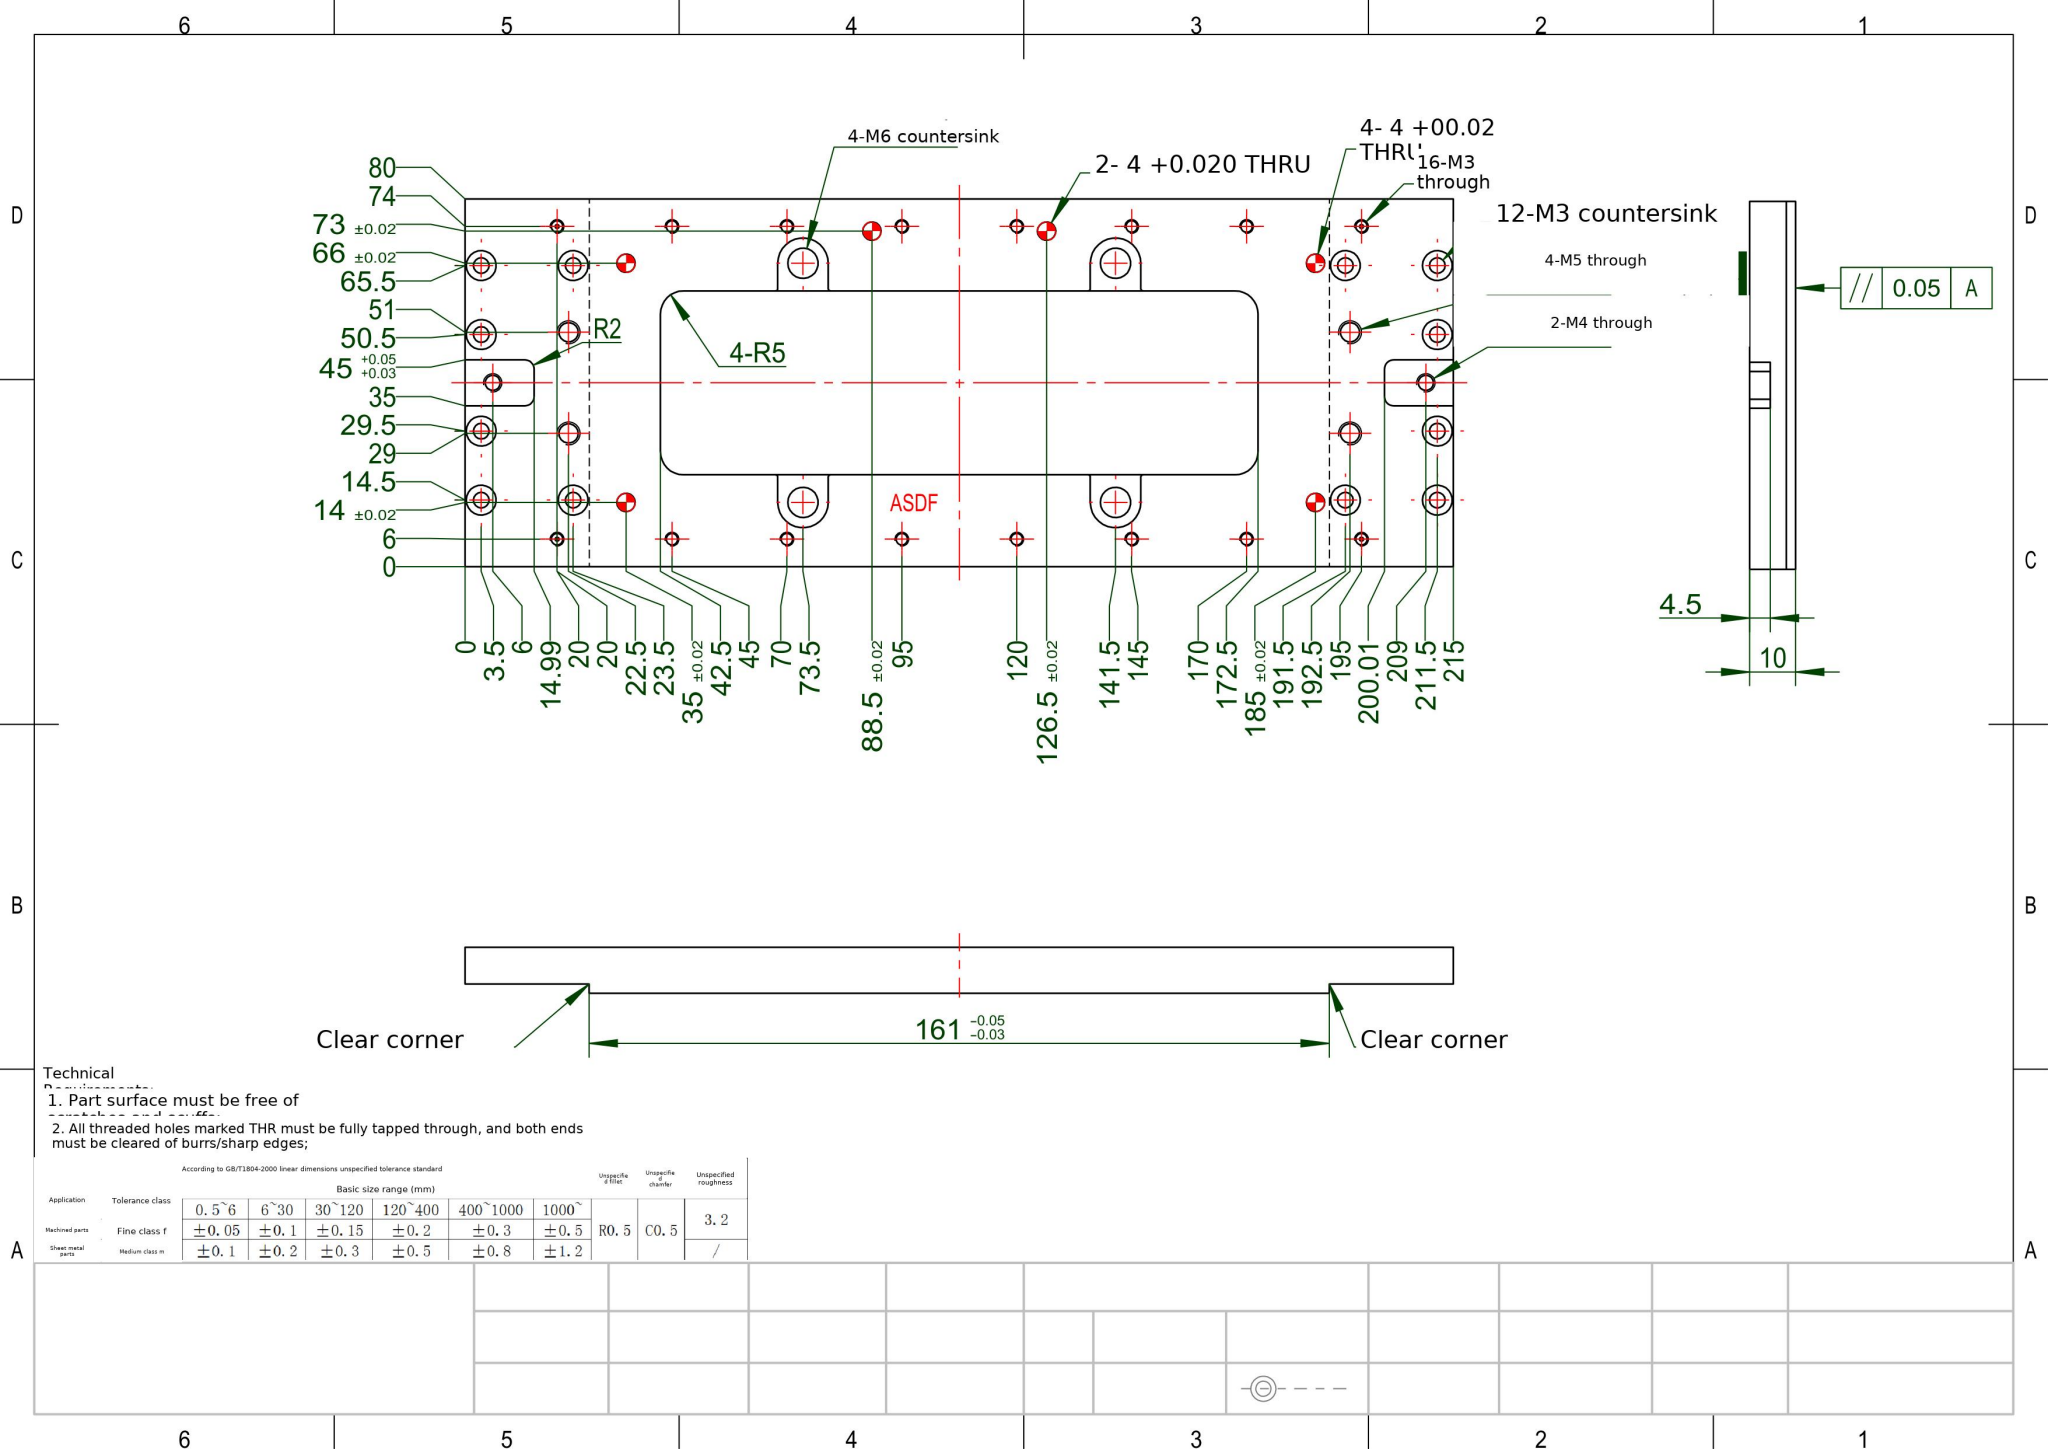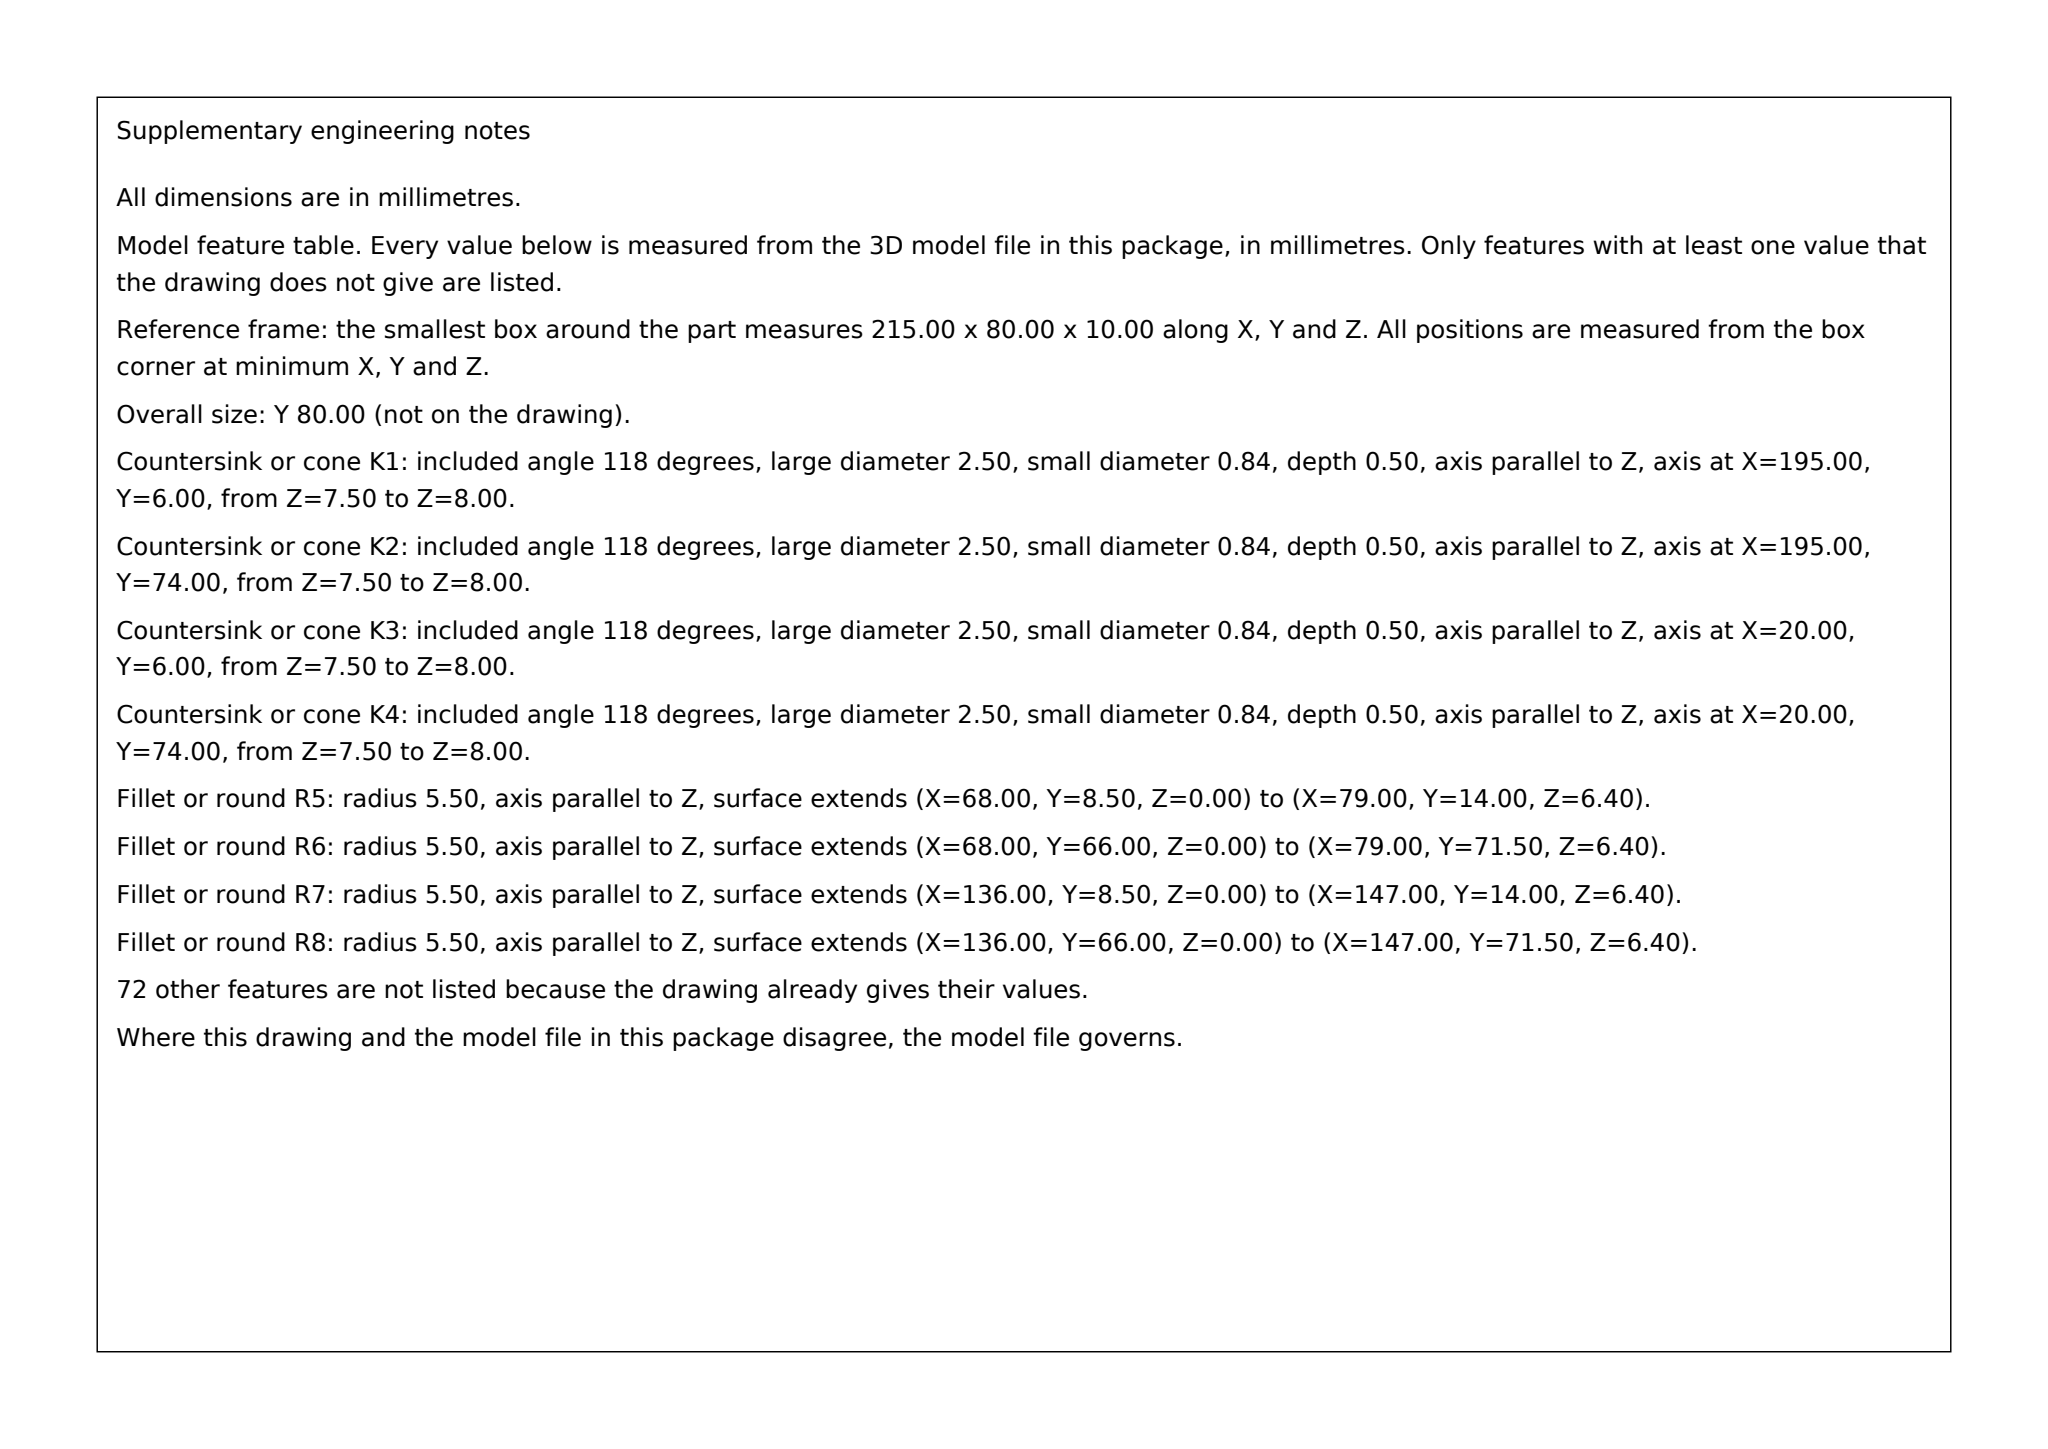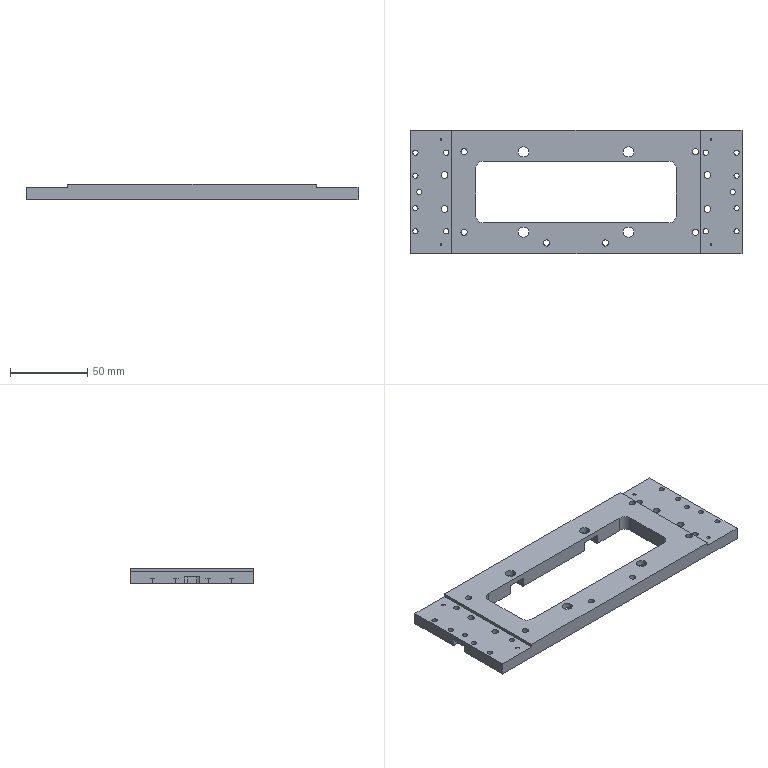Part | SolidWorks | mm | 1 solid | 210 faces | box 215 x 80 x 10 mm | volume 103119 mm3 | cylinder 132 | plane 46 | cone 32 | commonest cylinder face diameters 2.5 x32 6.5 x24 3.4 x24 4 x16 6.6 x8 4.2 x8 1 x8 3.3 x4